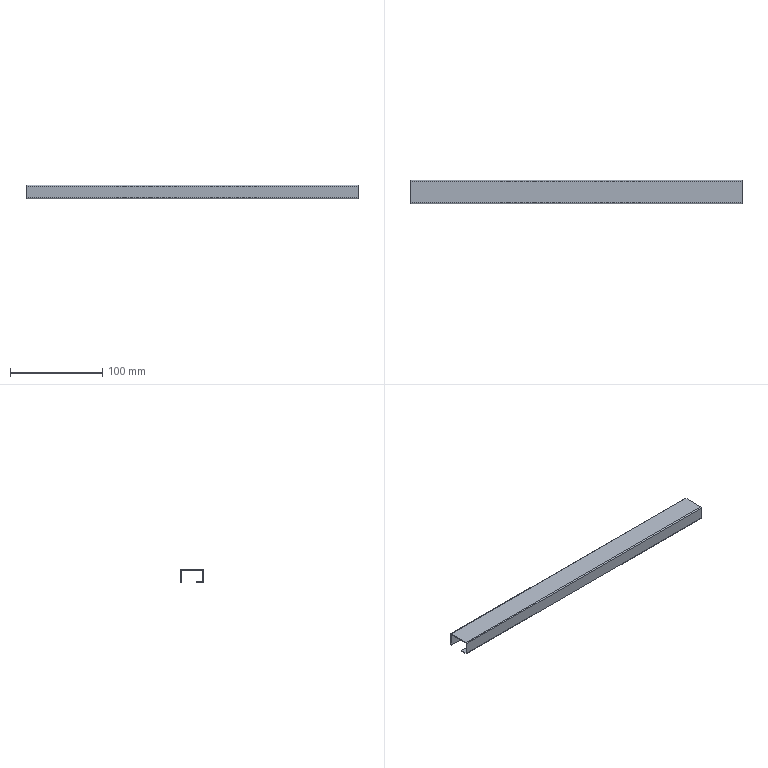Component | SolidWorks | MainBodyWeldment-1_MiddleBeam-1 | 1 solid | 30 faces | box 360 x 25 x 15 mm | volume 21322 mm3 | plane 24 | cylinder 6 | commonest cylinder face diameters 2.2 x3 0.2 x3 | material SPCC
STEP:
#1=CARTESIAN_POINT('',(6.938,7.278,9.295));
#2=VERTEX_POINT('',#1);
#3=CARTESIAN_POINT('',(6.938,7.318,9.295));
#4=VERTEX_POINT('',#3);
#5=CARTESIAN_POINT('',(6.938,7.278,9.295));
#6=DIRECTION('',(0.,1.,0.));
#7=VECTOR('',#6,39.37);
#8=LINE('',#5,#7);
#9=EDGE_CURVE('',#2,#4,#8,.T.);
#10=ORIENTED_EDGE('',*,*,#9,.F.);
#11=CARTESIAN_POINT('',(6.938,7.322,9.252));
#12=VERTEX_POINT('',#11);
#13=CARTESIAN_POINT('',(6.938,7.322,9.295));
#14=DIRECTION('',(-1.,0.,0.));
#15=DIRECTION('',(0.,0.,-1.));
#16=AXIS2_PLACEMENT_3D('',#13,#14,#15);
#17=CIRCLE('',#16,0.04331);
#18=EDGE_CURVE('',#12,#2,#17,.T.);
#19=ORIENTED_EDGE('',*,*,#18,.F.);
#20=CARTESIAN_POINT('',(6.938,7.322,9.291));
#21=VERTEX_POINT('',#20);
#22=CARTESIAN_POINT('',(6.938,7.322,9.291));
#23=DIRECTION('',(0.,0.,-1.));
#24=VECTOR('',#23,39.37);
#25=LINE('',#22,#24);
#26=EDGE_CURVE('',#21,#12,#25,.T.);
#27=ORIENTED_EDGE('',*,*,#26,.F.);
#28=CARTESIAN_POINT('',(6.938,7.322,9.295));
#29=DIRECTION('',(-1.,0.,0.));
#30=DIRECTION('',(0.,0.,-1.));
#31=AXIS2_PLACEMENT_3D('',#28,#29,#30);
#32=CIRCLE('',#31,0.003937);
#33=EDGE_CURVE('',#21,#4,#32,.T.);
#34=ORIENTED_EDGE('',*,*,#33,.T.);
#35=EDGE_LOOP('',(#10,#19,#27,#34));
#36=FACE_OUTER_BOUND('',#35,.T.);
#37=CARTESIAN_POINT('',(6.938,7.278,9.295));
#38=DIRECTION('',(1.,0.,0.));
#39=DIRECTION('',(0.,0.,-1.));
#40=AXIS2_PLACEMENT_3D('',#37,#38,#39);
#41=PLANE('',#40);
#42=ADVANCED_FACE('',(#36),#41,.T.);
#43=CARTESIAN_POINT('',(6.938,7.278,9.799));
#44=VERTEX_POINT('',#43);
#45=CARTESIAN_POINT('',(6.938,7.278,9.252));
#46=DIRECTION('',(0.,0.,1.));
#47=VECTOR('',#46,39.37);
#48=LINE('',#45,#47);
#49=EDGE_CURVE('',#2,#44,#48,.T.);
#50=ORIENTED_EDGE('',*,*,#49,.F.);
#51=ORIENTED_EDGE('',*,*,#9,.T.);
#52=CARTESIAN_POINT('',(6.938,7.318,9.799));
#53=VERTEX_POINT('',#52);
#54=CARTESIAN_POINT('',(6.938,7.318,9.252));
#55=DIRECTION('',(0.,0.,1.));
#56=VECTOR('',#55,39.37);
#57=LINE('',#54,#56);
#58=EDGE_CURVE('',#4,#53,#57,.T.);
#59=ORIENTED_EDGE('',*,*,#58,.T.);
#60=CARTESIAN_POINT('',(6.938,7.318,9.799));
#61=DIRECTION('',(0.,-1.,0.));
#62=VECTOR('',#61,39.37);
#63=LINE('',#60,#62);
#64=EDGE_CURVE('',#53,#44,#63,.T.);
#65=ORIENTED_EDGE('',*,*,#64,.T.);
#66=EDGE_LOOP('',(#50,#51,#59,#65));
#67=FACE_OUTER_BOUND('',#66,.T.);
#68=CARTESIAN_POINT('',(6.938,7.322,9.291));
#69=DIRECTION('',(1.,0.,0.));
#70=DIRECTION('',(0.,0.,-1.));
#71=AXIS2_PLACEMENT_3D('',#68,#69,#70);
#72=PLANE('',#71);
#73=ADVANCED_FACE('',(#67),#72,.T.);
#74=CARTESIAN_POINT('',(-7.236,7.322,9.252));
#75=VERTEX_POINT('',#74);
#76=CARTESIAN_POINT('',(-7.236,7.322,9.291));
#77=VERTEX_POINT('',#76);
#78=CARTESIAN_POINT('',(-7.236,7.322,9.252));
#79=DIRECTION('',(0.,0.,1.));
#80=VECTOR('',#79,39.37);
#81=LINE('',#78,#80);
#82=EDGE_CURVE('',#75,#77,#81,.T.);
#83=ORIENTED_EDGE('',*,*,#82,.F.);
#84=CARTESIAN_POINT('',(-7.236,7.278,9.295));
#85=VERTEX_POINT('',#84);
#86=CARTESIAN_POINT('',(-7.236,7.322,9.295));
#87=DIRECTION('',(-1.,0.,0.));
#88=DIRECTION('',(0.,0.,-1.));
#89=AXIS2_PLACEMENT_3D('',#86,#87,#88);
#90=CIRCLE('',#89,0.04331);
#91=EDGE_CURVE('',#75,#85,#90,.T.);
#92=ORIENTED_EDGE('',*,*,#91,.T.);
#93=CARTESIAN_POINT('',(-7.236,7.318,9.295));
#94=VERTEX_POINT('',#93);
#95=CARTESIAN_POINT('',(-7.236,7.318,9.295));
#96=DIRECTION('',(0.,-1.,0.));
#97=VECTOR('',#96,39.37);
#98=LINE('',#95,#97);
#99=EDGE_CURVE('',#94,#85,#98,.T.);
#100=ORIENTED_EDGE('',*,*,#99,.F.);
#101=CARTESIAN_POINT('',(-7.236,7.322,9.295));
#102=DIRECTION('',(-1.,0.,0.));
#103=DIRECTION('',(0.,0.,-1.));
#104=AXIS2_PLACEMENT_3D('',#101,#102,#103);
#105=CIRCLE('',#104,0.003937);
#106=EDGE_CURVE('',#77,#94,#105,.T.);
#107=ORIENTED_EDGE('',*,*,#106,.F.);
#108=EDGE_LOOP('',(#83,#92,#100,#107));
#109=FACE_OUTER_BOUND('',#108,.T.);
#110=CARTESIAN_POINT('',(-7.236,7.322,9.252));
#111=DIRECTION('',(-1.,0.,0.));
#112=DIRECTION('',(0.,0.,1.));
#113=AXIS2_PLACEMENT_3D('',#110,#111,#112);
#114=PLANE('',#113);
#115=ADVANCED_FACE('',(#109),#114,.T.);
#116=CARTESIAN_POINT('',(-7.236,7.593,9.252));
#117=VERTEX_POINT('',#116);
#118=CARTESIAN_POINT('',(-7.236,7.593,9.252));
#119=DIRECTION('',(0.,-1.,-0.));
#120=VECTOR('',#119,39.37);
#121=LINE('',#118,#120);
#122=EDGE_CURVE('',#117,#75,#121,.T.);
#123=ORIENTED_EDGE('',*,*,#122,.T.);
#124=ORIENTED_EDGE('',*,*,#82,.T.);
#125=CARTESIAN_POINT('',(-7.236,7.593,9.291));
#126=VERTEX_POINT('',#125);
#127=CARTESIAN_POINT('',(-7.236,7.593,9.291));
#128=DIRECTION('',(0.,-1.,-0.));
#129=VECTOR('',#128,39.37);
#130=LINE('',#127,#129);
#131=EDGE_CURVE('',#126,#77,#130,.T.);
#132=ORIENTED_EDGE('',*,*,#131,.F.);
#133=CARTESIAN_POINT('',(-7.236,7.593,9.291));
#134=DIRECTION('',(0.,0.,-1.));
#135=VECTOR('',#134,39.37);
#136=LINE('',#133,#135);
#137=EDGE_CURVE('',#126,#117,#136,.T.);
#138=ORIENTED_EDGE('',*,*,#137,.T.);
#139=EDGE_LOOP('',(#123,#124,#132,#138));
#140=FACE_OUTER_BOUND('',#139,.T.);
#141=CARTESIAN_POINT('',(-7.236,7.318,9.295));
#142=DIRECTION('',(-1.,0.,0.));
#143=DIRECTION('',(0.,0.,1.));
#144=AXIS2_PLACEMENT_3D('',#141,#142,#143);
#145=PLANE('',#144);
#146=ADVANCED_FACE('',(#140),#145,.T.);
#147=CARTESIAN_POINT('',(6.938,7.322,9.843));
#148=VERTEX_POINT('',#147);
#149=CARTESIAN_POINT('',(6.938,7.322,9.803));
#150=VERTEX_POINT('',#149);
#151=CARTESIAN_POINT('',(6.938,7.322,9.843));
#152=DIRECTION('',(0.,0.,-1.));
#153=VECTOR('',#152,39.37);
#154=LINE('',#151,#153);
#155=EDGE_CURVE('',#148,#150,#154,.T.);
#156=ORIENTED_EDGE('',*,*,#155,.F.);
#157=CARTESIAN_POINT('',(6.938,7.322,9.799));
#158=DIRECTION('',(-1.,0.,0.));
#159=DIRECTION('',(0.,0.,-1.));
#160=AXIS2_PLACEMENT_3D('',#157,#158,#159);
#161=CIRCLE('',#160,0.04331);
#162=EDGE_CURVE('',#44,#148,#161,.T.);
#163=ORIENTED_EDGE('',*,*,#162,.F.);
#164=ORIENTED_EDGE('',*,*,#64,.F.);
#165=CARTESIAN_POINT('',(6.938,7.322,9.799));
#166=DIRECTION('',(-1.,0.,0.));
#167=DIRECTION('',(0.,0.,-1.));
#168=AXIS2_PLACEMENT_3D('',#165,#166,#167);
#169=CIRCLE('',#168,0.003937);
#170=EDGE_CURVE('',#53,#150,#169,.T.);
#171=ORIENTED_EDGE('',*,*,#170,.T.);
#172=EDGE_LOOP('',(#156,#163,#164,#171));
#173=FACE_OUTER_BOUND('',#172,.T.);
#174=CARTESIAN_POINT('',(6.938,7.322,9.843));
#175=DIRECTION('',(1.,0.,0.));
#176=DIRECTION('',(0.,0.,-1.));
#177=AXIS2_PLACEMENT_3D('',#174,#175,#176);
#178=PLANE('',#177);
#179=ADVANCED_FACE('',(#173),#178,.T.);
#180=CARTESIAN_POINT('',(6.938,8.219,9.843));
#181=VERTEX_POINT('',#180);
#182=CARTESIAN_POINT('',(6.938,7.278,9.843));
#183=DIRECTION('',(0.,1.,0.));
#184=VECTOR('',#183,39.37);
#185=LINE('',#182,#184);
#186=EDGE_CURVE('',#148,#181,#185,.T.);
#187=ORIENTED_EDGE('',*,*,#186,.F.);
#188=ORIENTED_EDGE('',*,*,#155,.T.);
#189=CARTESIAN_POINT('',(6.938,8.219,9.803));
#190=VERTEX_POINT('',#189);
#191=CARTESIAN_POINT('',(6.938,7.278,9.803));
#192=DIRECTION('',(0.,1.,0.));
#193=VECTOR('',#192,39.37);
#194=LINE('',#191,#193);
#195=EDGE_CURVE('',#150,#190,#194,.T.);
#196=ORIENTED_EDGE('',*,*,#195,.T.);
#197=CARTESIAN_POINT('',(6.938,8.219,9.803));
#198=DIRECTION('',(0.,0.,1.));
#199=VECTOR('',#198,39.37);
#200=LINE('',#197,#199);
#201=EDGE_CURVE('',#190,#181,#200,.T.);
#202=ORIENTED_EDGE('',*,*,#201,.T.);
#203=EDGE_LOOP('',(#187,#188,#196,#202));
#204=FACE_OUTER_BOUND('',#203,.T.);
#205=CARTESIAN_POINT('',(6.938,7.318,9.799));
#206=DIRECTION('',(1.,0.,0.));
#207=DIRECTION('',(0.,0.,-1.));
#208=AXIS2_PLACEMENT_3D('',#205,#206,#207);
#209=PLANE('',#208);
#210=ADVANCED_FACE('',(#204),#209,.T.);
#211=CARTESIAN_POINT('',(-7.236,7.278,9.799));
#212=VERTEX_POINT('',#211);
#213=CARTESIAN_POINT('',(-7.236,7.318,9.799));
#214=VERTEX_POINT('',#213);
#215=CARTESIAN_POINT('',(-7.236,7.278,9.799));
#216=DIRECTION('',(0.,1.,0.));
#217=VECTOR('',#216,39.37);
#218=LINE('',#215,#217);
#219=EDGE_CURVE('',#212,#214,#218,.T.);
#220=ORIENTED_EDGE('',*,*,#219,.F.);
#221=CARTESIAN_POINT('',(-7.236,7.322,9.843));
#222=VERTEX_POINT('',#221);
#223=CARTESIAN_POINT('',(-7.236,7.322,9.799));
#224=DIRECTION('',(-1.,0.,0.));
#225=DIRECTION('',(0.,0.,-1.));
#226=AXIS2_PLACEMENT_3D('',#223,#224,#225);
#227=CIRCLE('',#226,0.04331);
#228=EDGE_CURVE('',#212,#222,#227,.T.);
#229=ORIENTED_EDGE('',*,*,#228,.T.);
#230=CARTESIAN_POINT('',(-7.236,7.322,9.803));
#231=VERTEX_POINT('',#230);
#232=CARTESIAN_POINT('',(-7.236,7.322,9.803));
#233=DIRECTION('',(0.,0.,1.));
#234=VECTOR('',#233,39.37);
#235=LINE('',#232,#234);
#236=EDGE_CURVE('',#231,#222,#235,.T.);
#237=ORIENTED_EDGE('',*,*,#236,.F.);
#238=CARTESIAN_POINT('',(-7.236,7.322,9.799));
#239=DIRECTION('',(-1.,0.,0.));
#240=DIRECTION('',(0.,0.,-1.));
#241=AXIS2_PLACEMENT_3D('',#238,#239,#240);
#242=CIRCLE('',#241,0.003937);
#243=EDGE_CURVE('',#214,#231,#242,.T.);
#244=ORIENTED_EDGE('',*,*,#243,.F.);
#245=EDGE_LOOP('',(#220,#229,#237,#244));
#246=FACE_OUTER_BOUND('',#245,.T.);
#247=CARTESIAN_POINT('',(-7.236,7.278,9.799));
#248=DIRECTION('',(-1.,0.,0.));
#249=DIRECTION('',(0.,0.,1.));
#250=AXIS2_PLACEMENT_3D('',#247,#248,#249);
#251=PLANE('',#250);
#252=ADVANCED_FACE('',(#246),#251,.T.);
#253=CARTESIAN_POINT('',(-7.236,7.278,9.252));
#254=DIRECTION('',(0.,0.,1.));
#255=VECTOR('',#254,39.37);
#256=LINE('',#253,#255);
#257=EDGE_CURVE('',#85,#212,#256,.T.);
#258=ORIENTED_EDGE('',*,*,#257,.T.);
#259=ORIENTED_EDGE('',*,*,#219,.T.);
#260=CARTESIAN_POINT('',(-7.236,7.318,9.252));
#261=DIRECTION('',(0.,0.,1.));
#262=VECTOR('',#261,39.37);
#263=LINE('',#260,#262);
#264=EDGE_CURVE('',#94,#214,#263,.T.);
#265=ORIENTED_EDGE('',*,*,#264,.F.);
#266=ORIENTED_EDGE('',*,*,#99,.T.);
#267=EDGE_LOOP('',(#258,#259,#265,#266));
#268=FACE_OUTER_BOUND('',#267,.T.);
#269=CARTESIAN_POINT('',(-7.236,7.322,9.803));
#270=DIRECTION('',(-1.,0.,0.));
#271=DIRECTION('',(0.,0.,1.));
#272=AXIS2_PLACEMENT_3D('',#269,#270,#271);
#273=PLANE('',#272);
#274=ADVANCED_FACE('',(#268),#273,.T.);
#275=CARTESIAN_POINT('',(6.938,8.263,9.799));
#276=VERTEX_POINT('',#275);
#277=CARTESIAN_POINT('',(6.938,8.223,9.799));
#278=VERTEX_POINT('',#277);
#279=CARTESIAN_POINT('',(6.938,8.263,9.799));
#280=DIRECTION('',(0.,-1.,0.));
#281=VECTOR('',#280,39.37);
#282=LINE('',#279,#281);
#283=EDGE_CURVE('',#276,#278,#282,.T.);
#284=ORIENTED_EDGE('',*,*,#283,.F.);
#285=CARTESIAN_POINT('',(6.938,8.219,9.799));
#286=DIRECTION('',(-1.,0.,0.));
#287=DIRECTION('',(0.,0.,-1.));
#288=AXIS2_PLACEMENT_3D('',#285,#286,#287);
#289=CIRCLE('',#288,0.04331);
#290=EDGE_CURVE('',#181,#276,#289,.T.);
#291=ORIENTED_EDGE('',*,*,#290,.F.);
#292=ORIENTED_EDGE('',*,*,#201,.F.);
#293=CARTESIAN_POINT('',(6.938,8.219,9.799));
#294=DIRECTION('',(-1.,0.,0.));
#295=DIRECTION('',(0.,0.,-1.));
#296=AXIS2_PLACEMENT_3D('',#293,#294,#295);
#297=CIRCLE('',#296,0.003937);
#298=EDGE_CURVE('',#190,#278,#297,.T.);
#299=ORIENTED_EDGE('',*,*,#298,.T.);
#300=EDGE_LOOP('',(#284,#291,#292,#299));
#301=FACE_OUTER_BOUND('',#300,.T.);
#302=CARTESIAN_POINT('',(6.938,8.263,9.799));
#303=DIRECTION('',(1.,0.,0.));
#304=DIRECTION('',(0.,0.,-1.));
#305=AXIS2_PLACEMENT_3D('',#302,#303,#304);
#306=PLANE('',#305);
#307=ADVANCED_FACE('',(#301),#306,.T.);
#308=CARTESIAN_POINT('',(6.938,8.263,9.252));
#309=VERTEX_POINT('',#308);
#310=CARTESIAN_POINT('',(6.938,8.263,9.843));
#311=DIRECTION('',(0.,0.,-1.));
#312=VECTOR('',#311,39.37);
#313=LINE('',#310,#312);
#314=EDGE_CURVE('',#276,#309,#313,.T.);
#315=ORIENTED_EDGE('',*,*,#314,.F.);
#316=ORIENTED_EDGE('',*,*,#283,.T.);
#317=CARTESIAN_POINT('',(6.938,8.223,9.252));
#318=VERTEX_POINT('',#317);
#319=CARTESIAN_POINT('',(6.938,8.223,9.843));
#320=DIRECTION('',(0.,0.,-1.));
#321=VECTOR('',#320,39.37);
#322=LINE('',#319,#321);
#323=EDGE_CURVE('',#278,#318,#322,.T.);
#324=ORIENTED_EDGE('',*,*,#323,.T.);
#325=CARTESIAN_POINT('',(6.938,8.263,9.252));
#326=DIRECTION('',(0.,-1.,0.));
#327=VECTOR('',#326,39.37);
#328=LINE('',#325,#327);
#329=EDGE_CURVE('',#309,#318,#328,.T.);
#330=ORIENTED_EDGE('',*,*,#329,.F.);
#331=EDGE_LOOP('',(#315,#316,#324,#330));
#332=FACE_OUTER_BOUND('',#331,.T.);
#333=CARTESIAN_POINT('',(6.938,8.219,9.803));
#334=DIRECTION('',(1.,0.,0.));
#335=DIRECTION('',(0.,0.,-1.));
#336=AXIS2_PLACEMENT_3D('',#333,#334,#335);
#337=PLANE('',#336);
#338=ADVANCED_FACE('',(#332),#337,.T.);
#339=CARTESIAN_POINT('',(-7.236,8.219,9.843));
#340=VERTEX_POINT('',#339);
#341=CARTESIAN_POINT('',(-7.236,8.219,9.803));
#342=VERTEX_POINT('',#341);
#343=CARTESIAN_POINT('',(-7.236,8.219,9.843));
#344=DIRECTION('',(0.,0.,-1.));
#345=VECTOR('',#344,39.37);
#346=LINE('',#343,#345);
#347=EDGE_CURVE('',#340,#342,#346,.T.);
#348=ORIENTED_EDGE('',*,*,#347,.F.);
#349=CARTESIAN_POINT('',(-7.236,8.263,9.799));
#350=VERTEX_POINT('',#349);
#351=CARTESIAN_POINT('',(-7.236,8.219,9.799));
#352=DIRECTION('',(-1.,0.,0.));
#353=DIRECTION('',(0.,0.,-1.));
#354=AXIS2_PLACEMENT_3D('',#351,#352,#353);
#355=CIRCLE('',#354,0.04331);
#356=EDGE_CURVE('',#340,#350,#355,.T.);
#357=ORIENTED_EDGE('',*,*,#356,.T.);
#358=CARTESIAN_POINT('',(-7.236,8.223,9.799));
#359=VERTEX_POINT('',#358);
#360=CARTESIAN_POINT('',(-7.236,8.223,9.799));
#361=DIRECTION('',(0.,1.,0.));
#362=VECTOR('',#361,39.37);
#363=LINE('',#360,#362);
#364=EDGE_CURVE('',#359,#350,#363,.T.);
#365=ORIENTED_EDGE('',*,*,#364,.F.);
#366=CARTESIAN_POINT('',(-7.236,8.219,9.799));
#367=DIRECTION('',(-1.,0.,0.));
#368=DIRECTION('',(0.,0.,-1.));
#369=AXIS2_PLACEMENT_3D('',#366,#367,#368);
#370=CIRCLE('',#369,0.003937);
#371=EDGE_CURVE('',#342,#359,#370,.T.);
#372=ORIENTED_EDGE('',*,*,#371,.F.);
#373=EDGE_LOOP('',(#348,#357,#365,#372));
#374=FACE_OUTER_BOUND('',#373,.T.);
#375=CARTESIAN_POINT('',(-7.236,8.219,9.843));
#376=DIRECTION('',(-1.,0.,0.));
#377=DIRECTION('',(0.,0.,1.));
#378=AXIS2_PLACEMENT_3D('',#375,#376,#377);
#379=PLANE('',#378);
#380=ADVANCED_FACE('',(#374),#379,.T.);
#381=CARTESIAN_POINT('',(-7.236,7.278,9.843));
#382=DIRECTION('',(0.,1.,0.));
#383=VECTOR('',#382,39.37);
#384=LINE('',#381,#383);
#385=EDGE_CURVE('',#222,#340,#384,.T.);
#386=ORIENTED_EDGE('',*,*,#385,.T.);
#387=ORIENTED_EDGE('',*,*,#347,.T.);
#388=CARTESIAN_POINT('',(-7.236,7.278,9.803));
#389=DIRECTION('',(0.,1.,0.));
#390=VECTOR('',#389,39.37);
#391=LINE('',#388,#390);
#392=EDGE_CURVE('',#231,#342,#391,.T.);
#393=ORIENTED_EDGE('',*,*,#392,.F.);
#394=ORIENTED_EDGE('',*,*,#236,.T.);
#395=EDGE_LOOP('',(#386,#387,#393,#394));
#396=FACE_OUTER_BOUND('',#395,.T.);
#397=CARTESIAN_POINT('',(-7.236,8.223,9.799));
#398=DIRECTION('',(-1.,0.,0.));
#399=DIRECTION('',(0.,0.,1.));
#400=AXIS2_PLACEMENT_3D('',#397,#398,#399);
#401=PLANE('',#400);
#402=ADVANCED_FACE('',(#396),#401,.T.);
#403=CARTESIAN_POINT('',(-7.236,8.223,9.252));
#404=VERTEX_POINT('',#403);
#405=CARTESIAN_POINT('',(-7.236,8.223,9.843));
#406=DIRECTION('',(0.,0.,-1.));
#407=VECTOR('',#406,39.37);
#408=LINE('',#405,#407);
#409=EDGE_CURVE('',#359,#404,#408,.T.);
#410=ORIENTED_EDGE('',*,*,#409,.T.);
#411=CARTESIAN_POINT('',(6.938,8.223,9.252));
#412=DIRECTION('',(-1.,0.,0.));
#413=VECTOR('',#412,39.37);
#414=LINE('',#411,#413);
#415=EDGE_CURVE('',#318,#404,#414,.T.);
#416=ORIENTED_EDGE('',*,*,#415,.F.);
#417=ORIENTED_EDGE('',*,*,#323,.F.);
#418=CARTESIAN_POINT('',(6.938,8.223,9.799));
#419=DIRECTION('',(-1.,0.,0.));
#420=VECTOR('',#419,39.37);
#421=LINE('',#418,#420);
#422=EDGE_CURVE('',#278,#359,#421,.T.);
#423=ORIENTED_EDGE('',*,*,#422,.T.);
#424=EDGE_LOOP('',(#410,#416,#417,#423));
#425=FACE_OUTER_BOUND('',#424,.T.);
#426=CARTESIAN_POINT('',(6.938,8.223,9.843));
#427=DIRECTION('',(0.,1.,0.));
#428=DIRECTION('',(0.,0.,1.));
#429=AXIS2_PLACEMENT_3D('',#426,#427,#428);
#430=PLANE('',#429);
#431=ADVANCED_FACE('',(#425),#430,.F.);
#432=CARTESIAN_POINT('',(-7.236,8.263,9.252));
#433=VERTEX_POINT('',#432);
#434=CARTESIAN_POINT('',(-7.236,8.263,9.252));
#435=DIRECTION('',(0.,-1.,0.));
#436=VECTOR('',#435,39.37);
#437=LINE('',#434,#436);
#438=EDGE_CURVE('',#433,#404,#437,.T.);
#439=ORIENTED_EDGE('',*,*,#438,.F.);
#440=CARTESIAN_POINT('',(6.938,8.263,9.252));
#441=DIRECTION('',(-1.,0.,0.));
#442=VECTOR('',#441,39.37);
#443=LINE('',#440,#442);
#444=EDGE_CURVE('',#309,#433,#443,.T.);
#445=ORIENTED_EDGE('',*,*,#444,.F.);
#446=ORIENTED_EDGE('',*,*,#329,.T.);
#447=ORIENTED_EDGE('',*,*,#415,.T.);
#448=EDGE_LOOP('',(#439,#445,#446,#447));
#449=FACE_OUTER_BOUND('',#448,.T.);
#450=CARTESIAN_POINT('',(6.938,8.263,9.252));
#451=DIRECTION('',(0.,0.,-1.));
#452=DIRECTION('',(-1.,0.,0.));
#453=AXIS2_PLACEMENT_3D('',#450,#451,#452);
#454=PLANE('',#453);
#455=ADVANCED_FACE('',(#449),#454,.T.);
#456=CARTESIAN_POINT('',(-7.236,8.263,9.843));
#457=DIRECTION('',(0.,0.,-1.));
#458=VECTOR('',#457,39.37);
#459=LINE('',#456,#458);
#460=EDGE_CURVE('',#350,#433,#459,.T.);
#461=ORIENTED_EDGE('',*,*,#460,.F.);
#462=CARTESIAN_POINT('',(6.938,8.263,9.799));
#463=DIRECTION('',(-1.,0.,0.));
#464=VECTOR('',#463,39.37);
#465=LINE('',#462,#464);
#466=EDGE_CURVE('',#276,#350,#465,.T.);
#467=ORIENTED_EDGE('',*,*,#466,.F.);
#468=ORIENTED_EDGE('',*,*,#314,.T.);
#469=ORIENTED_EDGE('',*,*,#444,.T.);
#470=EDGE_LOOP('',(#461,#467,#468,#469));
#471=FACE_OUTER_BOUND('',#470,.T.);
#472=CARTESIAN_POINT('',(6.938,8.263,9.843));
#473=DIRECTION('',(0.,1.,0.));
#474=DIRECTION('',(0.,0.,1.));
#475=AXIS2_PLACEMENT_3D('',#472,#473,#474);
#476=PLANE('',#475);
#477=ADVANCED_FACE('',(#471),#476,.T.);
#478=ORIENTED_EDGE('',*,*,#356,.F.);
#479=CARTESIAN_POINT('',(6.938,8.219,9.843));
#480=DIRECTION('',(-1.,0.,0.));
#481=VECTOR('',#480,39.37);
#482=LINE('',#479,#481);
#483=EDGE_CURVE('',#181,#340,#482,.T.);
#484=ORIENTED_EDGE('',*,*,#483,.F.);
#485=ORIENTED_EDGE('',*,*,#290,.T.);
#486=ORIENTED_EDGE('',*,*,#466,.T.);
#487=EDGE_LOOP('',(#478,#484,#485,#486));
#488=FACE_OUTER_BOUND('',#487,.T.);
#489=CARTESIAN_POINT('',(6.938,8.219,9.799));
#490=DIRECTION('',(-1.,0.,0.));
#491=DIRECTION('',(0.,0.,1.));
#492=AXIS2_PLACEMENT_3D('',#489,#490,#491);
#493=CYLINDRICAL_SURFACE('',#492,0.04331);
#494=ADVANCED_FACE('',(#488),#493,.T.);
#495=ORIENTED_EDGE('',*,*,#385,.F.);
#496=CARTESIAN_POINT('',(6.938,7.322,9.843));
#497=DIRECTION('',(-1.,0.,0.));
#498=VECTOR('',#497,39.37);
#499=LINE('',#496,#498);
#500=EDGE_CURVE('',#148,#222,#499,.T.);
#501=ORIENTED_EDGE('',*,*,#500,.F.);
#502=ORIENTED_EDGE('',*,*,#186,.T.);
#503=ORIENTED_EDGE('',*,*,#483,.T.);
#504=EDGE_LOOP('',(#495,#501,#502,#503));
#505=FACE_OUTER_BOUND('',#504,.T.);
#506=CARTESIAN_POINT('',(6.938,7.278,9.843));
#507=DIRECTION('',(0.,0.,1.));
#508=DIRECTION('',(1.,0.,0.));
#509=AXIS2_PLACEMENT_3D('',#506,#507,#508);
#510=PLANE('',#509);
#511=ADVANCED_FACE('',(#505),#510,.T.);
#512=ORIENTED_EDGE('',*,*,#228,.F.);
#513=CARTESIAN_POINT('',(6.938,7.278,9.799));
#514=DIRECTION('',(-1.,0.,0.));
#515=VECTOR('',#514,39.37);
#516=LINE('',#513,#515);
#517=EDGE_CURVE('',#44,#212,#516,.T.);
#518=ORIENTED_EDGE('',*,*,#517,.F.);
#519=ORIENTED_EDGE('',*,*,#162,.T.);
#520=ORIENTED_EDGE('',*,*,#500,.T.);
#521=EDGE_LOOP('',(#512,#518,#519,#520));
#522=FACE_OUTER_BOUND('',#521,.T.);
#523=CARTESIAN_POINT('',(6.938,7.322,9.799));
#524=DIRECTION('',(-1.,0.,0.));
#525=DIRECTION('',(0.,0.,1.));
#526=AXIS2_PLACEMENT_3D('',#523,#524,#525);
#527=CYLINDRICAL_SURFACE('',#526,0.04331);
#528=ADVANCED_FACE('',(#522),#527,.T.);
#529=ORIENTED_EDGE('',*,*,#257,.F.);
#530=CARTESIAN_POINT('',(6.938,7.278,9.295));
#531=DIRECTION('',(-1.,0.,0.));
#532=VECTOR('',#531,39.37);
#533=LINE('',#530,#532);
#534=EDGE_CURVE('',#2,#85,#533,.T.);
#535=ORIENTED_EDGE('',*,*,#534,.F.);
#536=ORIENTED_EDGE('',*,*,#49,.T.);
#537=ORIENTED_EDGE('',*,*,#517,.T.);
#538=EDGE_LOOP('',(#529,#535,#536,#537));
#539=FACE_OUTER_BOUND('',#538,.T.);
#540=CARTESIAN_POINT('',(6.938,7.278,9.252));
#541=DIRECTION('',(0.,-1.,0.));
#542=DIRECTION('',(0.,-0.,-1.));
#543=AXIS2_PLACEMENT_3D('',#540,#541,#542);
#544=PLANE('',#543);
#545=ADVANCED_FACE('',(#539),#544,.T.);
#546=ORIENTED_EDGE('',*,*,#91,.F.);
#547=CARTESIAN_POINT('',(6.938,7.322,9.252));
#548=DIRECTION('',(-1.,0.,0.));
#549=VECTOR('',#548,39.37);
#550=LINE('',#547,#549);
#551=EDGE_CURVE('',#12,#75,#550,.T.);
#552=ORIENTED_EDGE('',*,*,#551,.F.);
#553=ORIENTED_EDGE('',*,*,#18,.T.);
#554=ORIENTED_EDGE('',*,*,#534,.T.);
#555=EDGE_LOOP('',(#546,#552,#553,#554));
#556=FACE_OUTER_BOUND('',#555,.T.);
#557=CARTESIAN_POINT('',(6.938,7.322,9.295));
#558=DIRECTION('',(-1.,0.,0.));
#559=DIRECTION('',(0.,0.,1.));
#560=AXIS2_PLACEMENT_3D('',#557,#558,#559);
#561=CYLINDRICAL_SURFACE('',#560,0.04331);
#562=ADVANCED_FACE('',(#556),#561,.T.);
#563=ORIENTED_EDGE('',*,*,#122,.F.);
#564=CARTESIAN_POINT('',(6.938,7.593,9.252));
#565=VERTEX_POINT('',#564);
#566=CARTESIAN_POINT('',(6.938,7.593,9.252));
#567=DIRECTION('',(-1.,0.,0.));
#568=VECTOR('',#567,39.37);
#569=LINE('',#566,#568);
#570=EDGE_CURVE('',#565,#117,#569,.T.);
#571=ORIENTED_EDGE('',*,*,#570,.F.);
#572=CARTESIAN_POINT('',(6.938,7.593,9.252));
#573=DIRECTION('',(0.,-1.,-0.));
#574=VECTOR('',#573,39.37);
#575=LINE('',#572,#574);
#576=EDGE_CURVE('',#565,#12,#575,.T.);
#577=ORIENTED_EDGE('',*,*,#576,.T.);
#578=ORIENTED_EDGE('',*,*,#551,.T.);
#579=EDGE_LOOP('',(#563,#571,#577,#578));
#580=FACE_OUTER_BOUND('',#579,.T.);
#581=CARTESIAN_POINT('',(6.938,7.593,9.252));
#582=DIRECTION('',(0.,0.,-1.));
#583=DIRECTION('',(0.,1.,0.));
#584=AXIS2_PLACEMENT_3D('',#581,#582,#583);
#585=PLANE('',#584);
#586=ADVANCED_FACE('',(#580),#585,.T.);
#587=ORIENTED_EDGE('',*,*,#137,.F.);
#588=CARTESIAN_POINT('',(6.938,7.593,9.291));
#589=VERTEX_POINT('',#588);
#590=CARTESIAN_POINT('',(6.938,7.593,9.291));
#591=DIRECTION('',(-1.,0.,0.));
#592=VECTOR('',#591,39.37);
#593=LINE('',#590,#592);
#594=EDGE_CURVE('',#589,#126,#593,.T.);
#595=ORIENTED_EDGE('',*,*,#594,.F.);
#596=CARTESIAN_POINT('',(6.938,7.593,9.291));
#597=DIRECTION('',(0.,0.,-1.));
#598=VECTOR('',#597,39.37);
#599=LINE('',#596,#598);
#600=EDGE_CURVE('',#589,#565,#599,.T.);
#601=ORIENTED_EDGE('',*,*,#600,.T.);
#602=ORIENTED_EDGE('',*,*,#570,.T.);
#603=EDGE_LOOP('',(#587,#595,#601,#602));
#604=FACE_OUTER_BOUND('',#603,.T.);
#605=CARTESIAN_POINT('',(6.938,7.593,9.291));
#606=DIRECTION('',(0.,1.,0.));
#607=DIRECTION('',(0.,0.,1.));
#608=AXIS2_PLACEMENT_3D('',#605,#606,#607);
#609=PLANE('',#608);
#610=ADVANCED_FACE('',(#604),#609,.T.);
#611=ORIENTED_EDGE('',*,*,#131,.T.);
#612=CARTESIAN_POINT('',(6.938,7.322,9.291));
#613=DIRECTION('',(-1.,0.,0.));
#614=VECTOR('',#613,39.37);
#615=LINE('',#612,#614);
#616=EDGE_CURVE('',#21,#77,#615,.T.);
#617=ORIENTED_EDGE('',*,*,#616,.F.);
#618=CARTESIAN_POINT('',(6.938,7.593,9.291));
#619=DIRECTION('',(0.,-1.,-0.));
#620=VECTOR('',#619,39.37);
#621=LINE('',#618,#620);
#622=EDGE_CURVE('',#589,#21,#621,.T.);
#623=ORIENTED_EDGE('',*,*,#622,.F.);
#624=ORIENTED_EDGE('',*,*,#594,.T.);
#625=EDGE_LOOP('',(#611,#617,#623,#624));
#626=FACE_OUTER_BOUND('',#625,.T.);
#627=CARTESIAN_POINT('',(6.938,7.593,9.291));
#628=DIRECTION('',(0.,0.,-1.));
#629=DIRECTION('',(0.,1.,0.));
#630=AXIS2_PLACEMENT_3D('',#627,#628,#629);
#631=PLANE('',#630);
#632=ADVANCED_FACE('',(#626),#631,.F.);
#633=ORIENTED_EDGE('',*,*,#106,.T.);
#634=CARTESIAN_POINT('',(6.938,7.318,9.295));
#635=DIRECTION('',(-1.,0.,0.));
#636=VECTOR('',#635,39.37);
#637=LINE('',#634,#636);
#638=EDGE_CURVE('',#4,#94,#637,.T.);
#639=ORIENTED_EDGE('',*,*,#638,.F.);
#640=ORIENTED_EDGE('',*,*,#33,.F.);
#641=ORIENTED_EDGE('',*,*,#616,.T.);
#642=EDGE_LOOP('',(#633,#639,#640,#641));
#643=FACE_OUTER_BOUND('',#642,.T.);
#644=CARTESIAN_POINT('',(6.938,7.322,9.295));
#645=DIRECTION('',(-1.,0.,0.));
#646=DIRECTION('',(0.,0.,1.));
#647=AXIS2_PLACEMENT_3D('',#644,#645,#646);
#648=CYLINDRICAL_SURFACE('',#647,0.003937);
#649=ADVANCED_FACE('',(#643),#648,.F.);
#650=ORIENTED_EDGE('',*,*,#264,.T.);
#651=CARTESIAN_POINT('',(6.938,7.318,9.799));
#652=DIRECTION('',(-1.,0.,0.));
#653=VECTOR('',#652,39.37);
#654=LINE('',#651,#653);
#655=EDGE_CURVE('',#53,#214,#654,.T.);
#656=ORIENTED_EDGE('',*,*,#655,.F.);
#657=ORIENTED_EDGE('',*,*,#58,.F.);
#658=ORIENTED_EDGE('',*,*,#638,.T.);
#659=EDGE_LOOP('',(#650,#656,#657,#658));
#660=FACE_OUTER_BOUND('',#659,.T.);
#661=CARTESIAN_POINT('',(6.938,7.318,9.252));
#662=DIRECTION('',(0.,-1.,0.));
#663=DIRECTION('',(0.,-0.,-1.));
#664=AXIS2_PLACEMENT_3D('',#661,#662,#663);
#665=PLANE('',#664);
#666=ADVANCED_FACE('',(#660),#665,.F.);
#667=ORIENTED_EDGE('',*,*,#243,.T.);
#668=CARTESIAN_POINT('',(6.938,7.322,9.803));
#669=DIRECTION('',(-1.,0.,0.));
#670=VECTOR('',#669,39.37);
#671=LINE('',#668,#670);
#672=EDGE_CURVE('',#150,#231,#671,.T.);
#673=ORIENTED_EDGE('',*,*,#672,.F.);
#674=ORIENTED_EDGE('',*,*,#170,.F.);
#675=ORIENTED_EDGE('',*,*,#655,.T.);
#676=EDGE_LOOP('',(#667,#673,#674,#675));
#677=FACE_OUTER_BOUND('',#676,.T.);
#678=CARTESIAN_POINT('',(6.938,7.322,9.799));
#679=DIRECTION('',(-1.,0.,0.));
#680=DIRECTION('',(0.,0.,1.));
#681=AXIS2_PLACEMENT_3D('',#678,#679,#680);
#682=CYLINDRICAL_SURFACE('',#681,0.003937);
#683=ADVANCED_FACE('',(#677),#682,.F.);
#684=ORIENTED_EDGE('',*,*,#392,.T.);
#685=CARTESIAN_POINT('',(6.938,8.219,9.803));
#686=DIRECTION('',(-1.,0.,0.));
#687=VECTOR('',#686,39.37);
#688=LINE('',#685,#687);
#689=EDGE_CURVE('',#190,#342,#688,.T.);
#690=ORIENTED_EDGE('',*,*,#689,.F.);
#691=ORIENTED_EDGE('',*,*,#195,.F.);
#692=ORIENTED_EDGE('',*,*,#672,.T.);
#693=EDGE_LOOP('',(#684,#690,#691,#692));
#694=FACE_OUTER_BOUND('',#693,.T.);
#695=CARTESIAN_POINT('',(6.938,7.278,9.803));
#696=DIRECTION('',(0.,0.,1.));
#697=DIRECTION('',(1.,0.,0.));
#698=AXIS2_PLACEMENT_3D('',#695,#696,#697);
#699=PLANE('',#698);
#700=ADVANCED_FACE('',(#694),#699,.F.);
#701=ORIENTED_EDGE('',*,*,#371,.T.);
#702=ORIENTED_EDGE('',*,*,#422,.F.);
#703=ORIENTED_EDGE('',*,*,#298,.F.);
#704=ORIENTED_EDGE('',*,*,#689,.T.);
#705=EDGE_LOOP('',(#701,#702,#703,#704));
#706=FACE_OUTER_BOUND('',#705,.T.);
#707=CARTESIAN_POINT('',(6.938,8.219,9.799));
#708=DIRECTION('',(-1.,0.,0.));
#709=DIRECTION('',(0.,0.,1.));
#710=AXIS2_PLACEMENT_3D('',#707,#708,#709);
#711=CYLINDRICAL_SURFACE('',#710,0.003937);
#712=ADVANCED_FACE('',(#706),#711,.F.);
#713=ORIENTED_EDGE('',*,*,#622,.T.);
#714=ORIENTED_EDGE('',*,*,#26,.T.);
#715=ORIENTED_EDGE('',*,*,#576,.F.);
#716=ORIENTED_EDGE('',*,*,#600,.F.);
#717=EDGE_LOOP('',(#713,#714,#715,#716));
#718=FACE_OUTER_BOUND('',#717,.T.);
#719=CARTESIAN_POINT('',(6.938,8.219,9.799));
#720=DIRECTION('',(1.,0.,0.));
#721=DIRECTION('',(0.,0.,-1.));
#722=AXIS2_PLACEMENT_3D('',#719,#720,#721);
#723=PLANE('',#722);
#724=ADVANCED_FACE('',(#718),#723,.T.);
#725=ORIENTED_EDGE('',*,*,#409,.F.);
#726=ORIENTED_EDGE('',*,*,#364,.T.);
#727=ORIENTED_EDGE('',*,*,#460,.T.);
#728=ORIENTED_EDGE('',*,*,#438,.T.);
#729=EDGE_LOOP('',(#725,#726,#727,#728));
#730=FACE_OUTER_BOUND('',#729,.T.);
#731=CARTESIAN_POINT('',(-7.236,8.219,9.799));
#732=DIRECTION('',(1.,0.,0.));
#733=DIRECTION('',(0.,0.,-1.));
#734=AXIS2_PLACEMENT_3D('',#731,#732,#733);
#735=PLANE('',#734);
#736=ADVANCED_FACE('',(#730),#735,.F.);
#737=CLOSED_SHELL('',(#42,#73,#115,#146,#179,#210,#252,#274,#307,#338,#380,#402,#431,#455,#477,#494,#511,#528,#545,#562,#586,#610,#632,#649,#666,#683,#700,#712,#724,#736));
#738=MANIFOLD_SOLID_BREP('',#737);
#739=CARTESIAN_POINT('',(0.,0.,0.));
#740=DIRECTION('',(0.,0.,1.));
#741=DIRECTION('',(1.,0.,0.));
#742=AXIS2_PLACEMENT_3D('',#739,#740,#741);
#743=(LENGTH_UNIT()NAMED_UNIT(*)SI_UNIT($,.METRE.));
#744=LENGTH_MEASURE_WITH_UNIT(LENGTH_MEASURE(0.0254),#743);
#745=DIMENSIONAL_EXPONENTS(1.,0.,0.,0.,0.,0.,0.);
#746=(CONVERSION_BASED_UNIT('',#744)LENGTH_UNIT()NAMED_UNIT(#745));
#747=UNCERTAINTY_MEASURE_WITH_UNIT(LENGTH_MEASURE(0.00001),#746,'','');
#748=(NAMED_UNIT(*)PLANE_ANGLE_UNIT()SI_UNIT($,.RADIAN.));
#749=(NAMED_UNIT(*)SI_UNIT($,.STERADIAN.)SOLID_ANGLE_UNIT());
#750=(GEOMETRIC_REPRESENTATION_CONTEXT(3)GLOBAL_UNCERTAINTY_ASSIGNED_CONTEXT((#747))GLOBAL_UNIT_ASSIGNED_CONTEXT((#746,#748,#749))REPRESENTATION_CONTEXT('',''));
#751=ADVANCED_BREP_SHAPE_REPRESENTATION('',(#738,#742),#750);
#752=COLOUR_RGB('',0.7922,0.8196,0.9333);
#753=FILL_AREA_STYLE_COLOUR('',#752);
#754=FILL_AREA_STYLE('',(#753));
#755=SURFACE_STYLE_FILL_AREA(#754);
#756=SURFACE_SIDE_STYLE('',(#755));
#757=SURFACE_STYLE_USAGE(.BOTH.,#756);
#758=PRESENTATION_STYLE_ASSIGNMENT((#757));
#759=STYLED_ITEM('',(#758),#738);
#760=(LENGTH_UNIT()NAMED_UNIT(*)SI_UNIT($,.METRE.));
#761=LENGTH_MEASURE_WITH_UNIT(LENGTH_MEASURE(0.0254),#760);
#762=DIMENSIONAL_EXPONENTS(1.,0.,0.,0.,0.,0.,0.);
#763=(CONVERSION_BASED_UNIT('',#761)LENGTH_UNIT()NAMED_UNIT(#762));
#764=UNCERTAINTY_MEASURE_WITH_UNIT(LENGTH_MEASURE(0.00001),#763,'','');
#765=(NAMED_UNIT(*)PLANE_ANGLE_UNIT()SI_UNIT($,.RADIAN.));
#766=(NAMED_UNIT(*)SI_UNIT($,.STERADIAN.)SOLID_ANGLE_UNIT());
#767=(GEOMETRIC_REPRESENTATION_CONTEXT(3)GLOBAL_UNCERTAINTY_ASSIGNED_CONTEXT((#764))GLOBAL_UNIT_ASSIGNED_CONTEXT((#763,#765,#766))REPRESENTATION_CONTEXT('',''));
#768=MECHANICAL_DESIGN_GEOMETRIC_PRESENTATION_REPRESENTATION('',(#759),#767);
#769=PRESENTATION_LAYER_ASSIGNMENT('','',(#759));